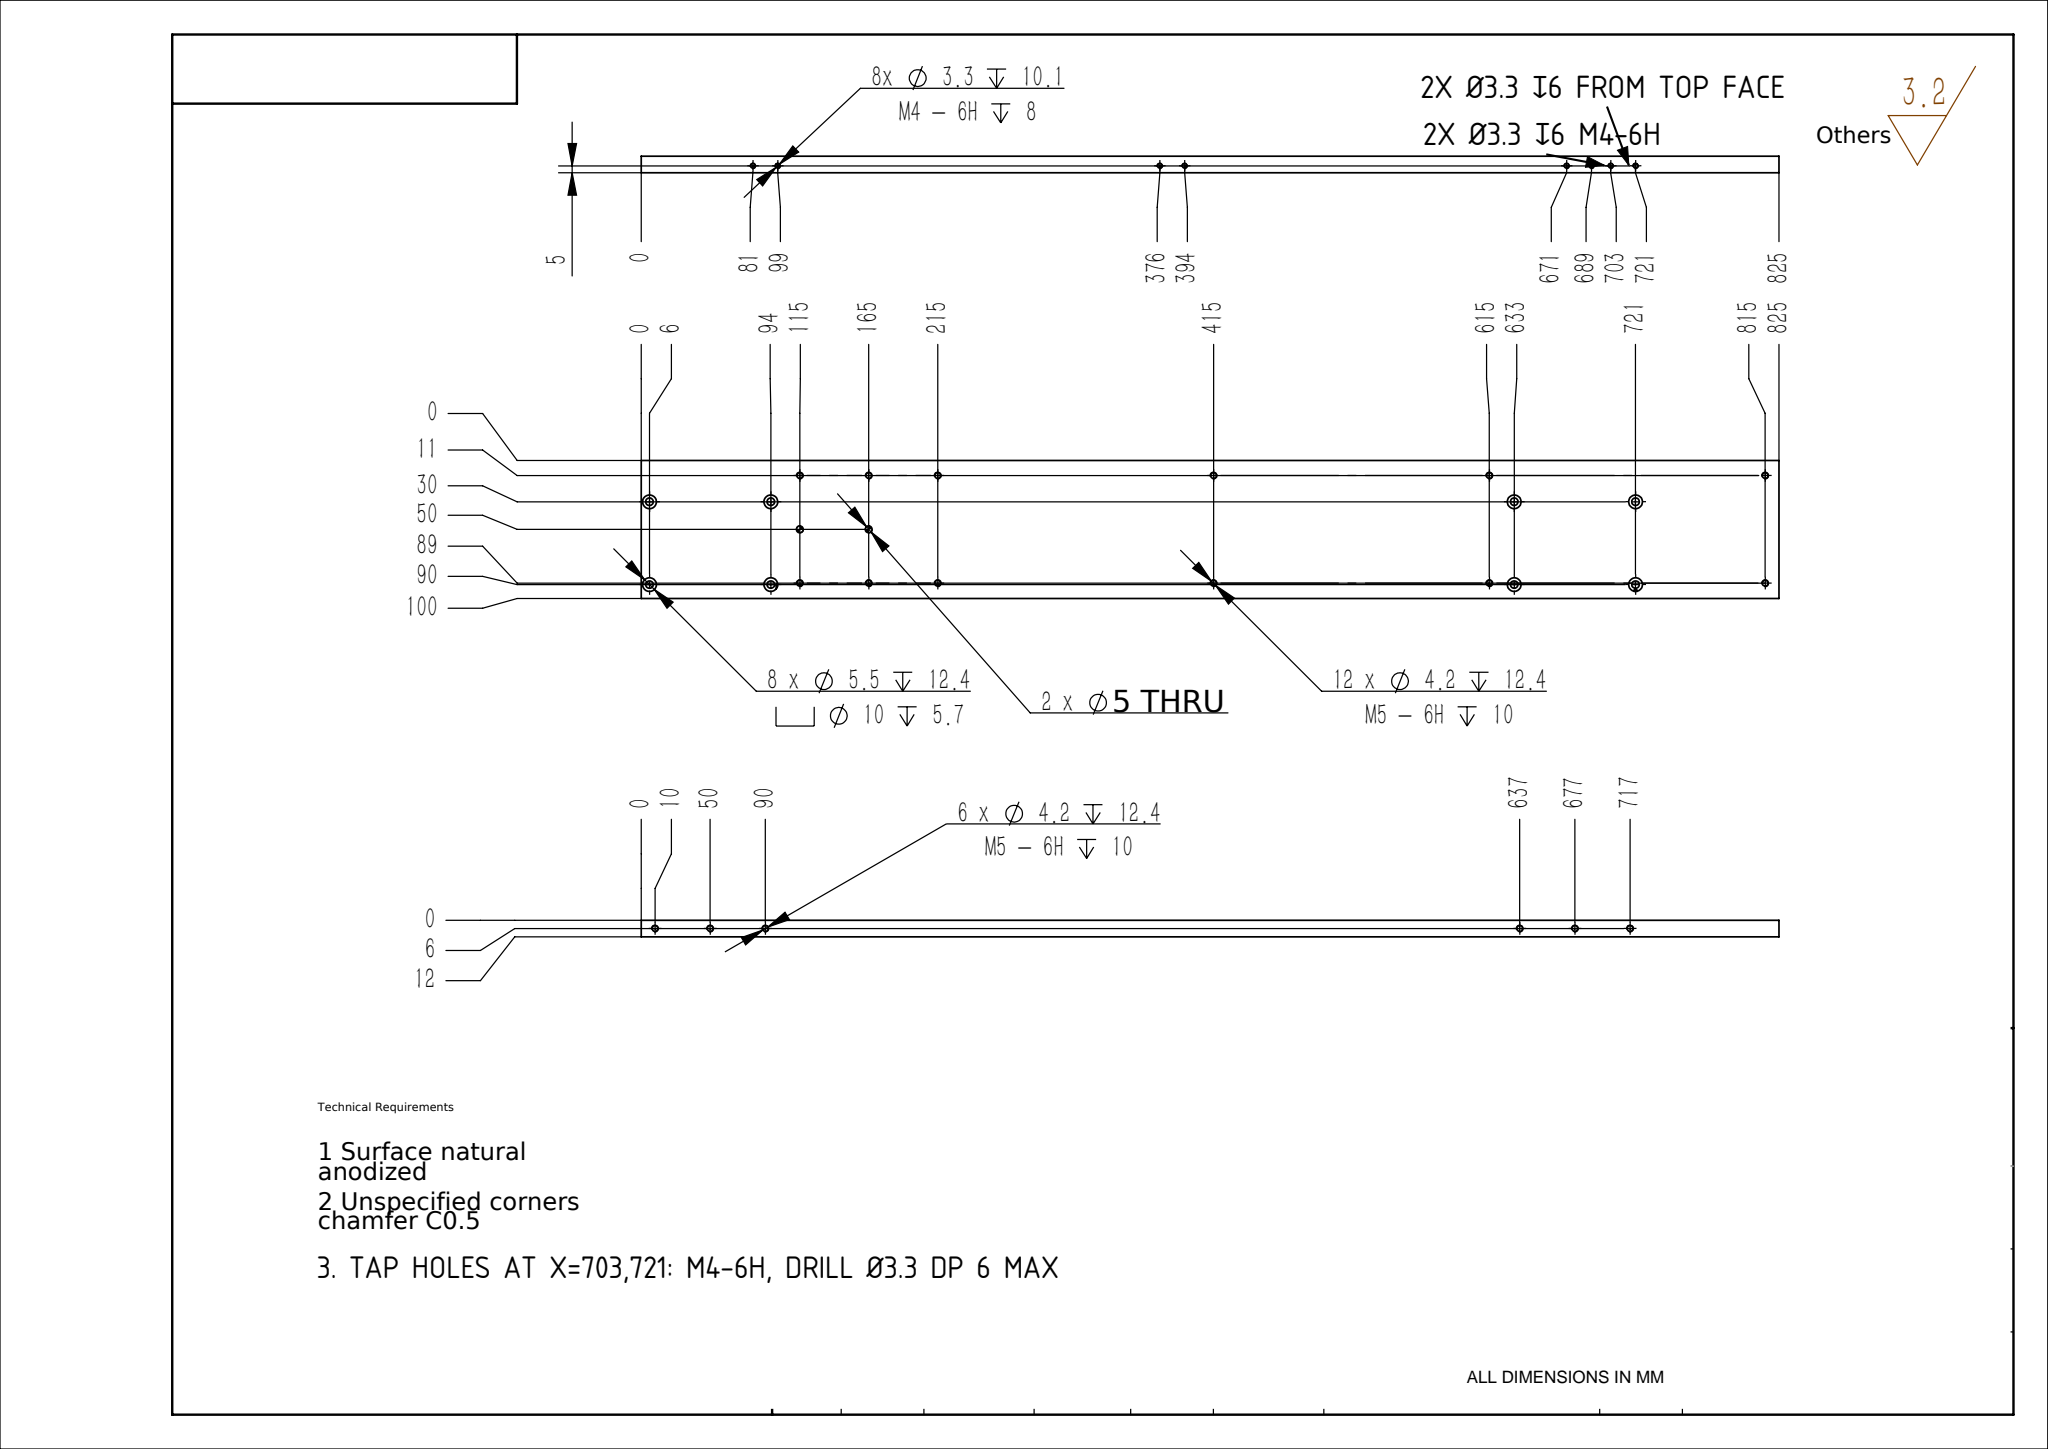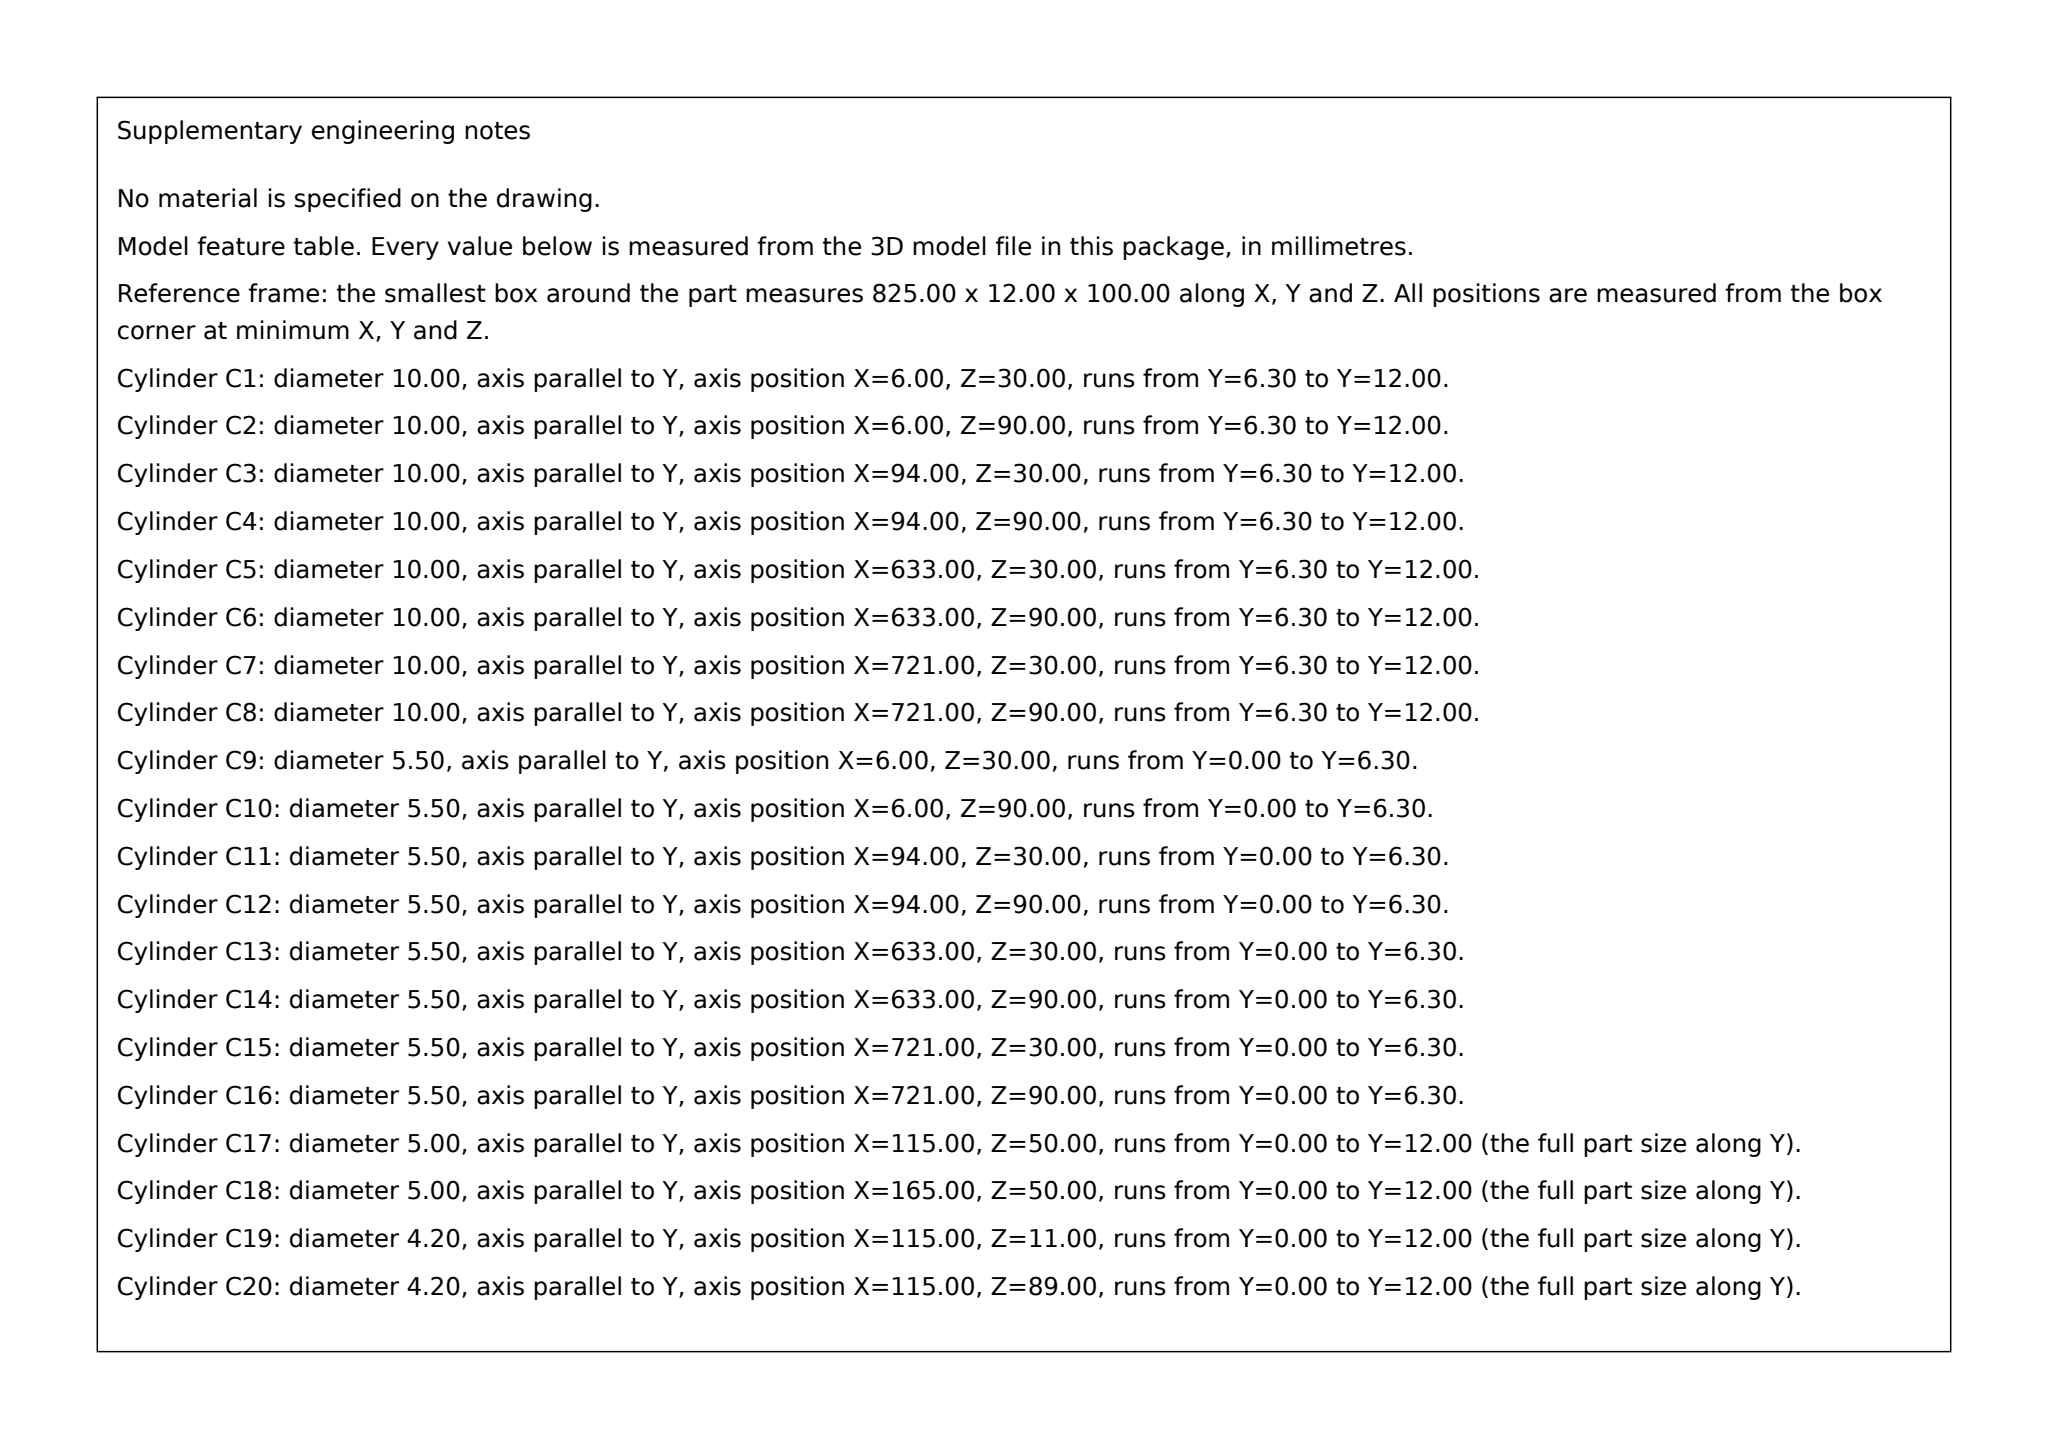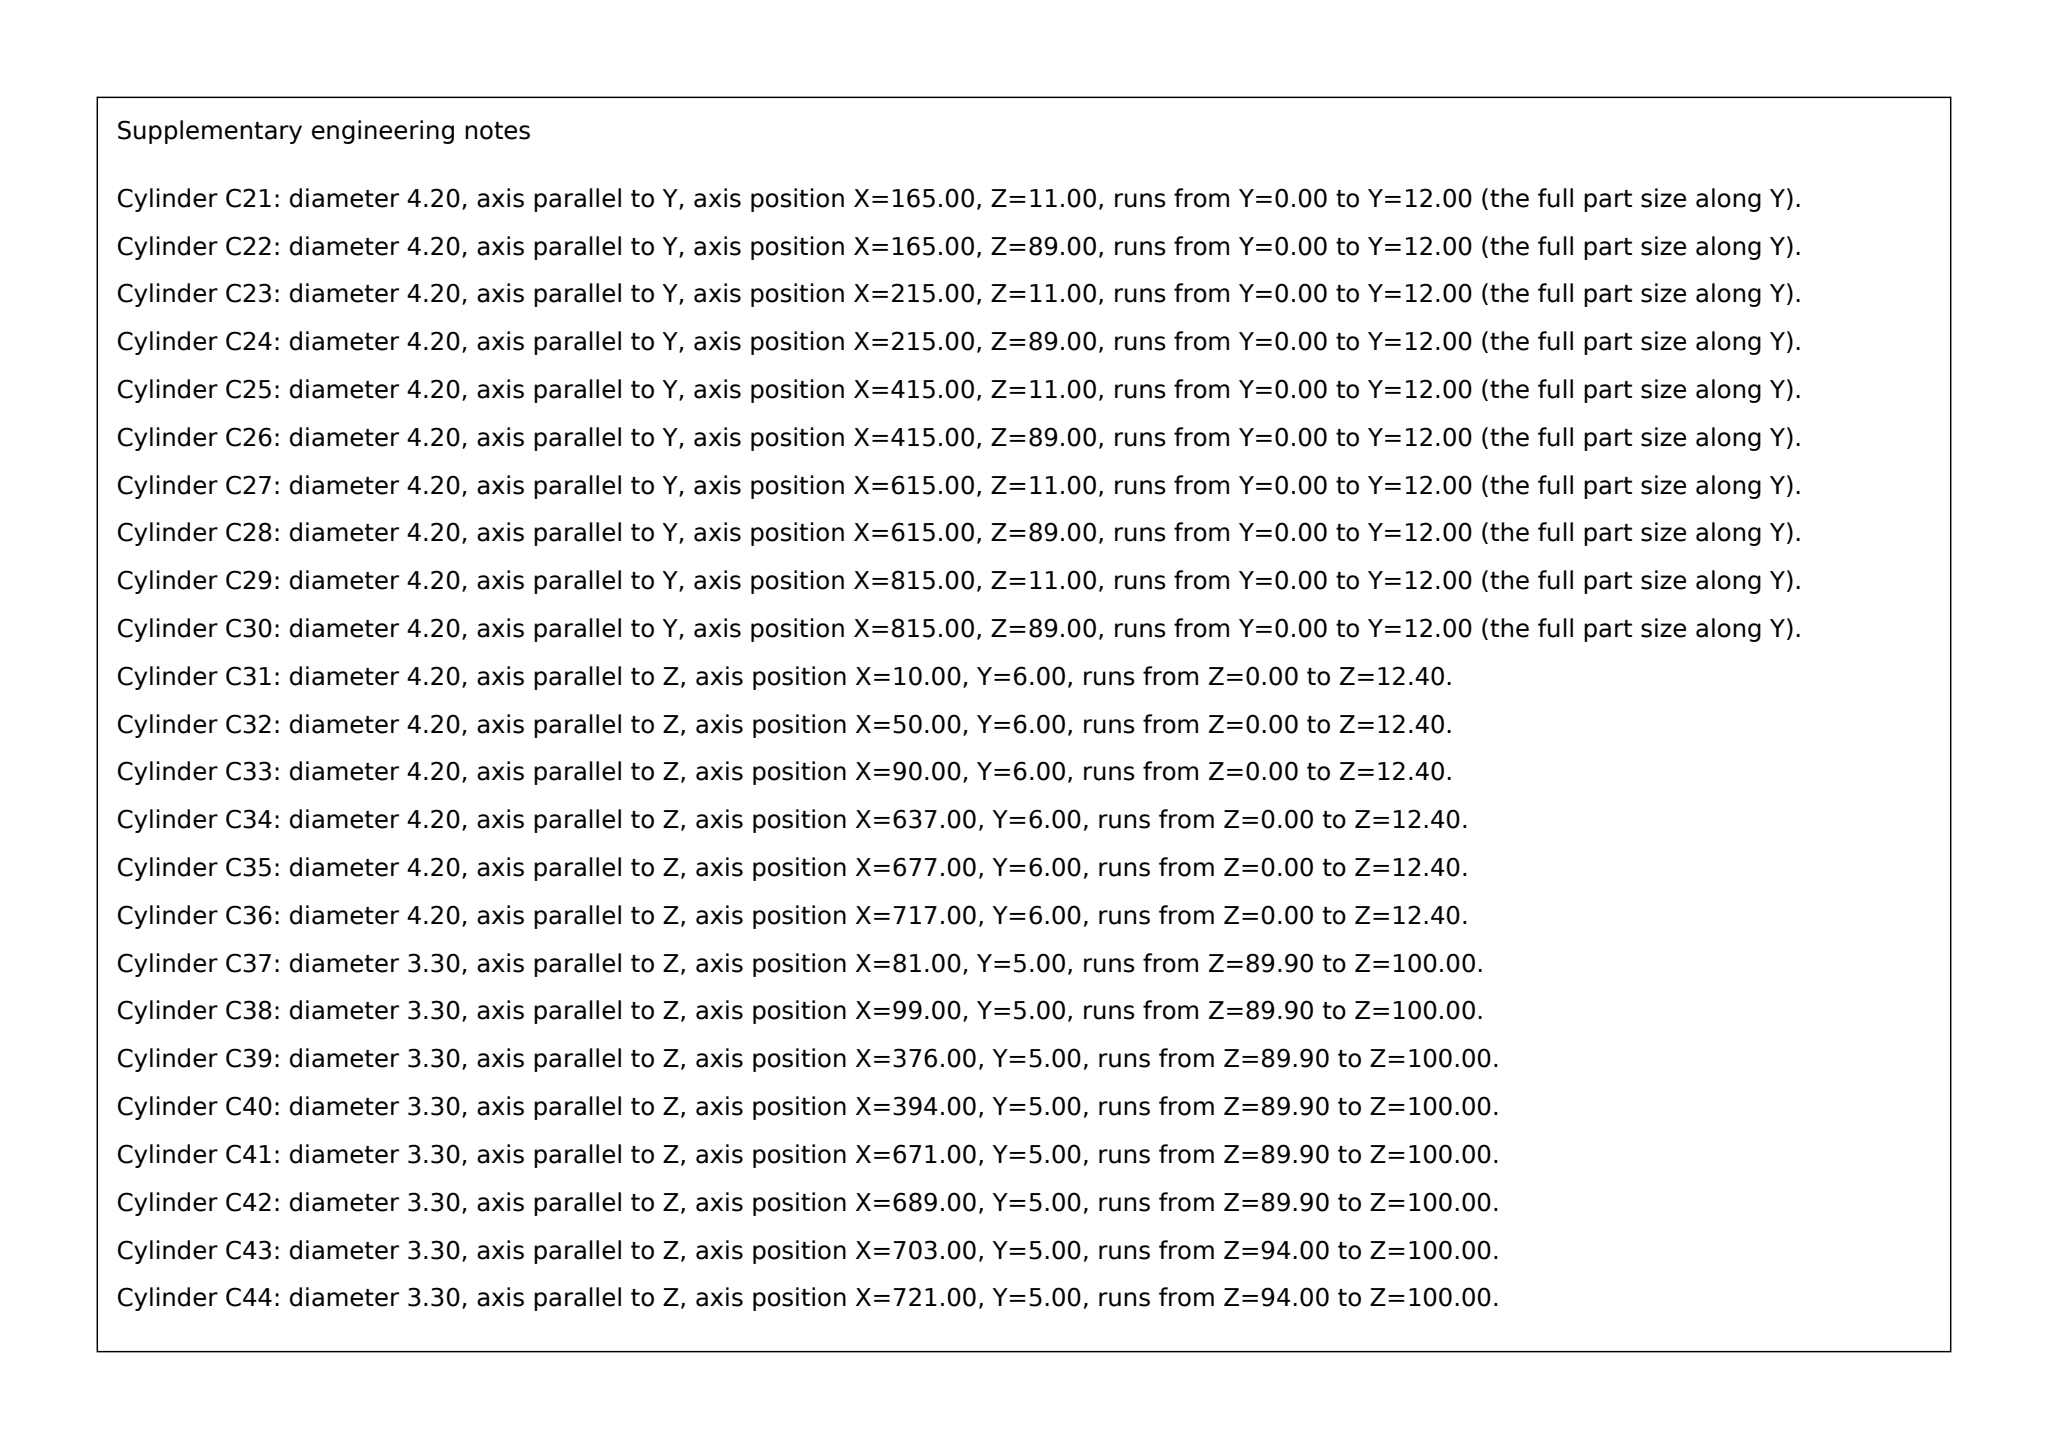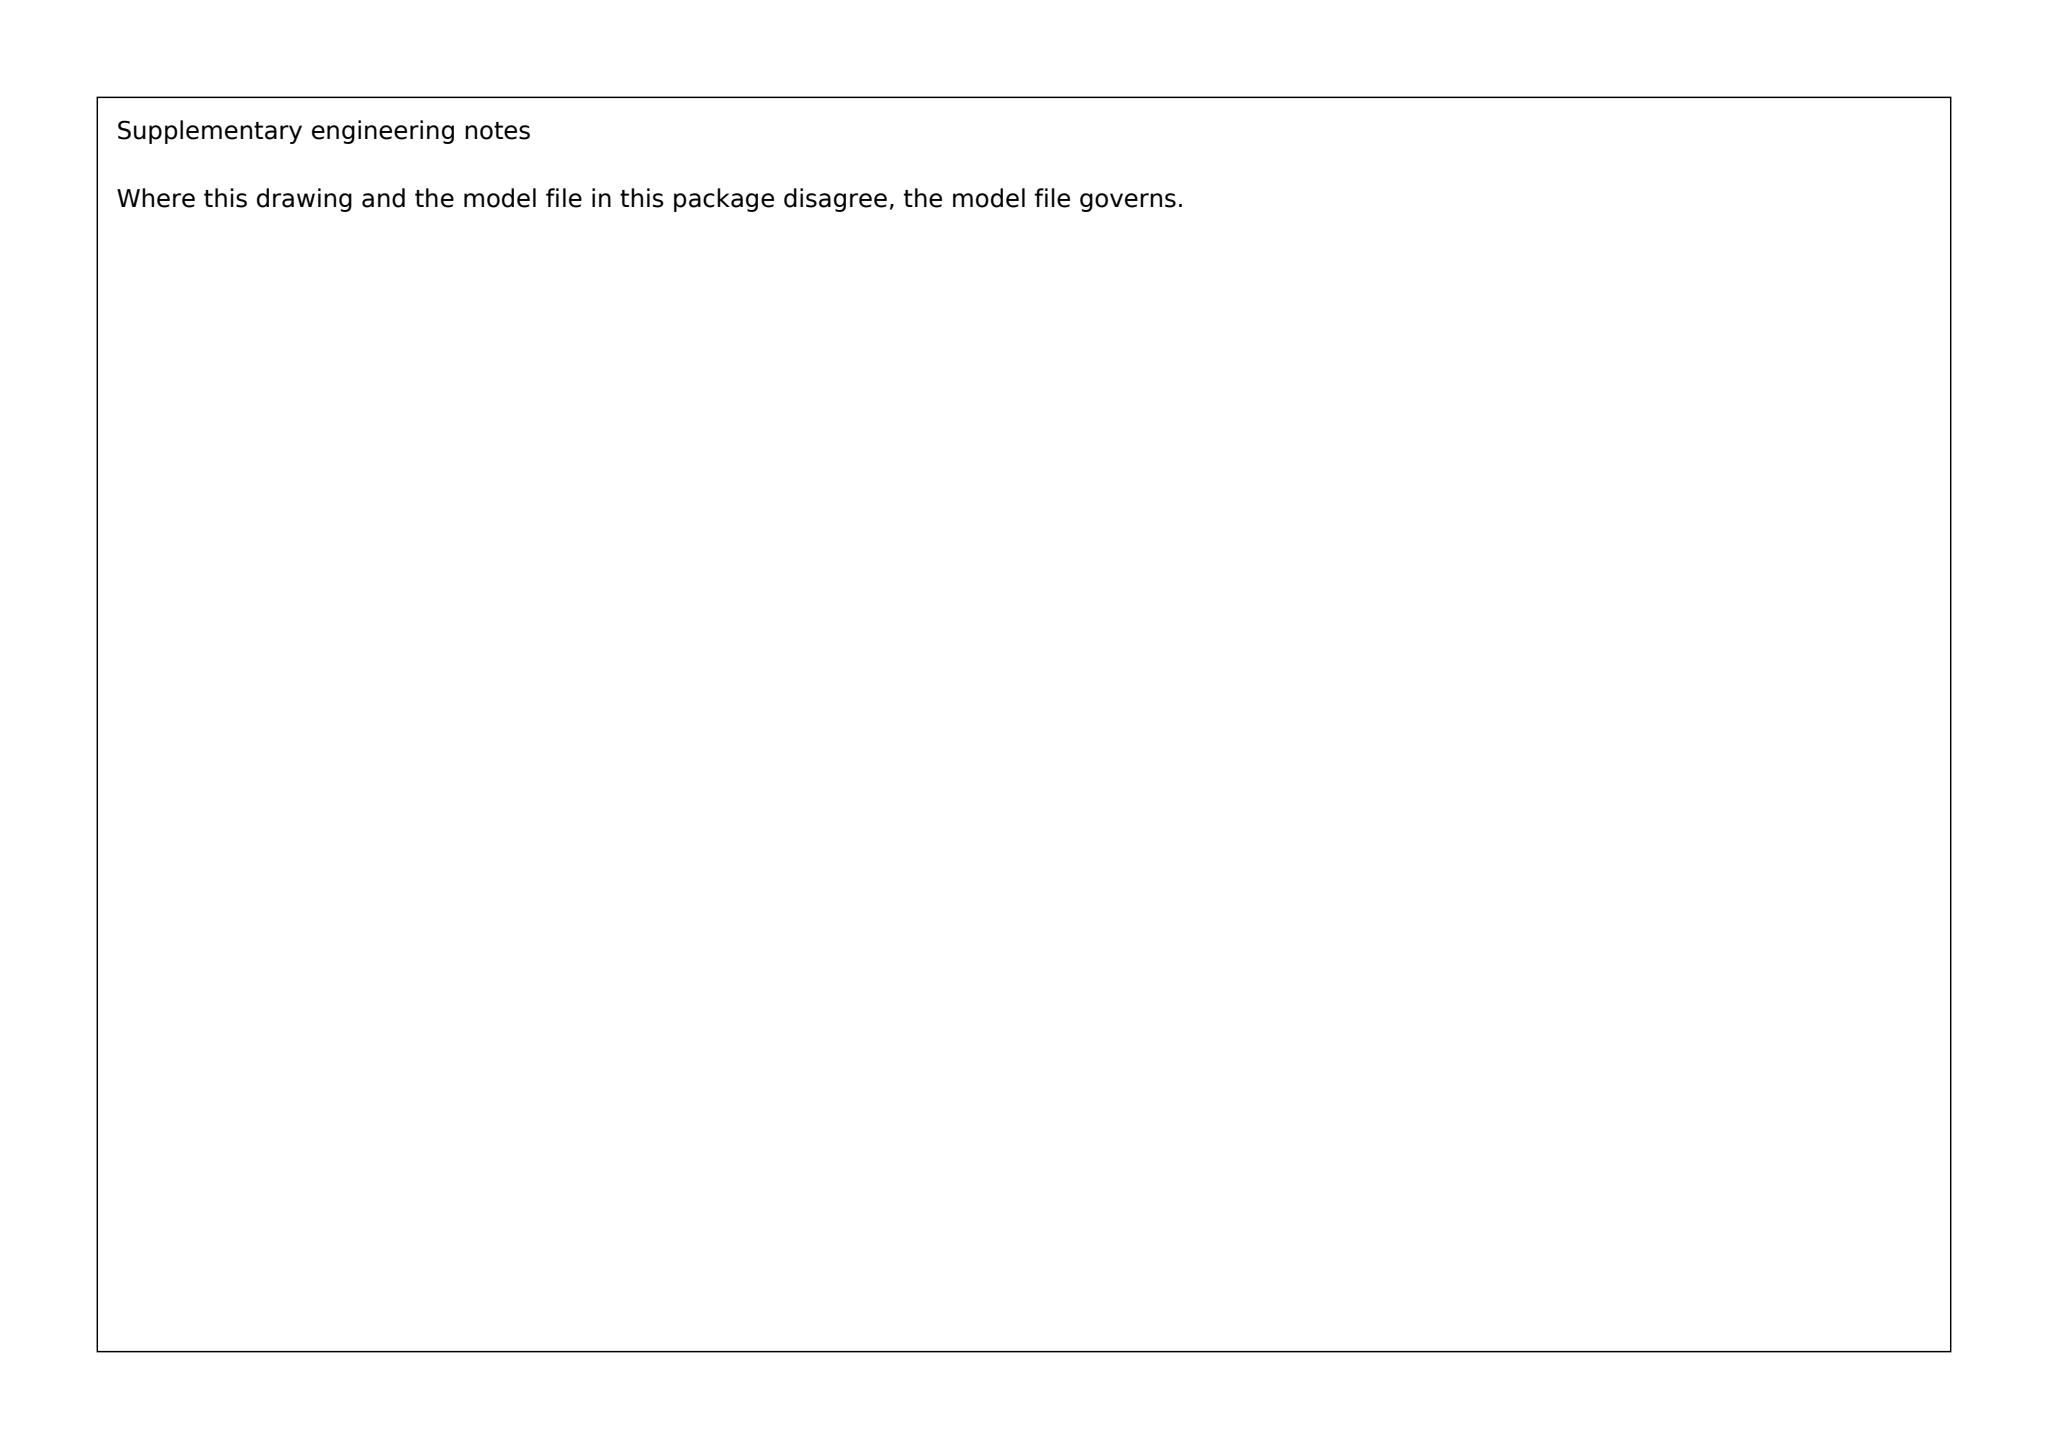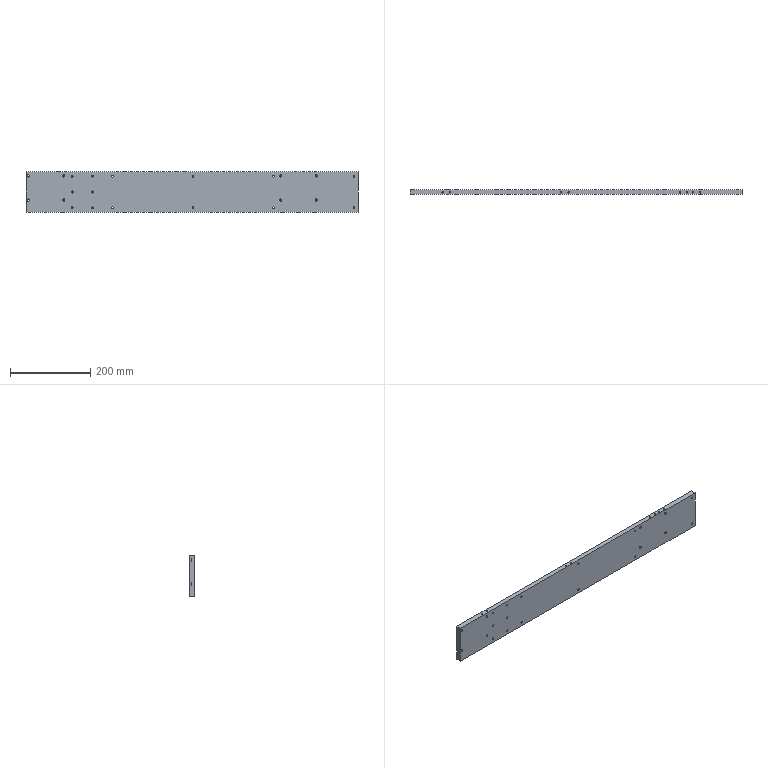Part | SolidWorks | mm | 1 solid | 130 faces | box 825 x 12 x 100 mm | volume 981047 mm3 | cylinder 88 | cone 28 | plane 14 | commonest cylinder face diameters 4.2 x36 3.3 x16 10 x16 5.5 x16 5 x4
Drawing notes:
2X Ø3.3 DP 6 (M4-6H) AT X=703 & 721, FROM TOP FACE | from the solid: Ø3.3 z-axis holes at x=703,721 span z=94.0→100.0 (6 deep) vs others 89.9→100.0
2X Ø3.3 DP 6 (DRILL DEPTH FROM TOP FACE) AT X=703 & 721 | from the solid: Ø3.3 z-holes at (703,5) & (721,5) run z=94.0 to 100.0 (top face z=100) => 6 deep; drill point cone to z=93.0
TAP HOLES AT X=703,721: M4-6H, DRILL Ø3.3 DP 6 MAX | from the solid: Only Ø3.3 full-dia depth 6.0 exists in STEP (z 94->100); no thread feature modeled